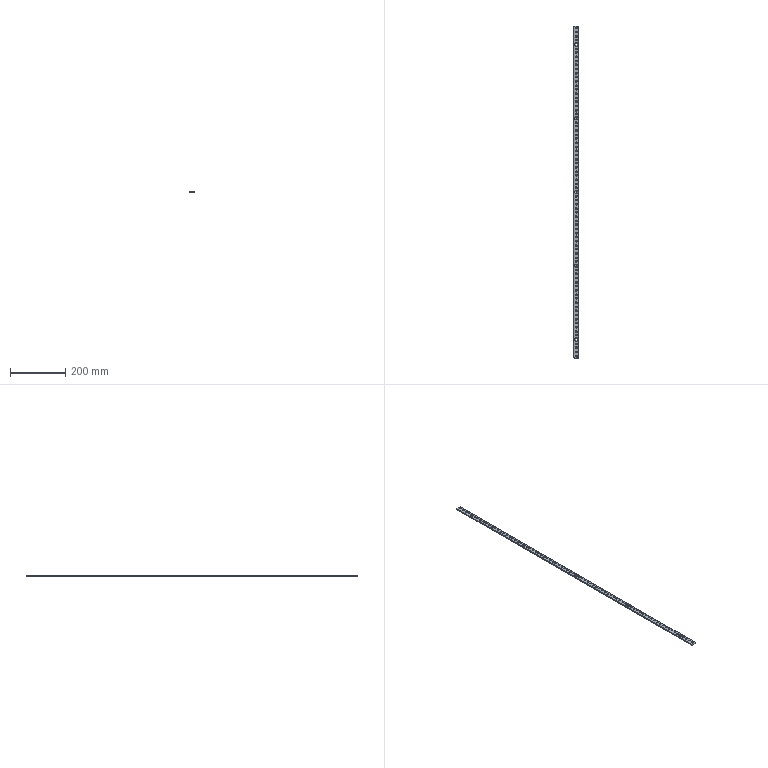CAM job | Mastercam | mm | 9 operations | part box 17.3 x 1200.15 x 6
1. Contour (Ramp) | 9 - 10 平铣刀
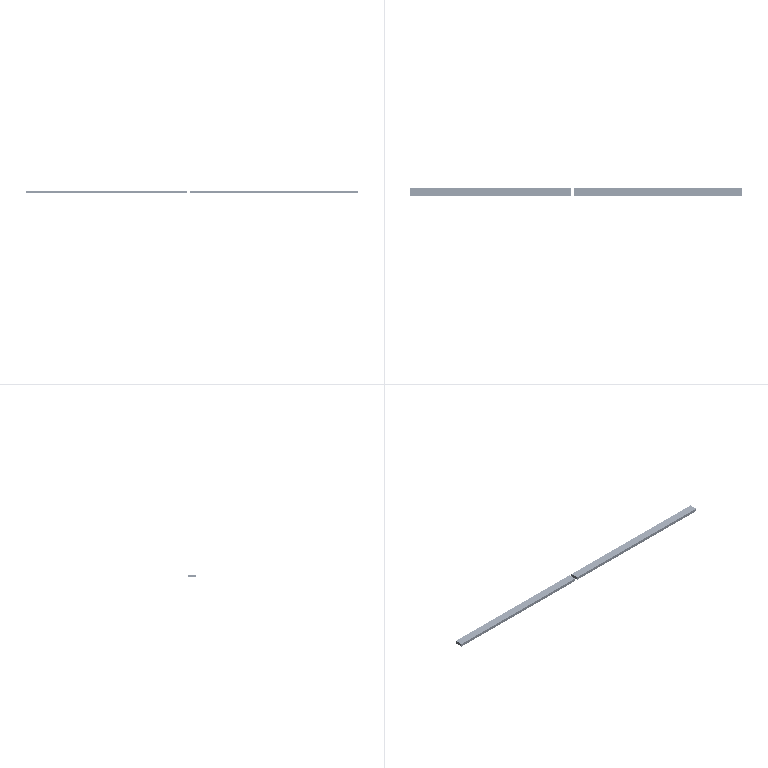2. Contour (2D) | 10 - 10 平铣刀
3. Drill/Counterbore | 7 - 6 倒角刀
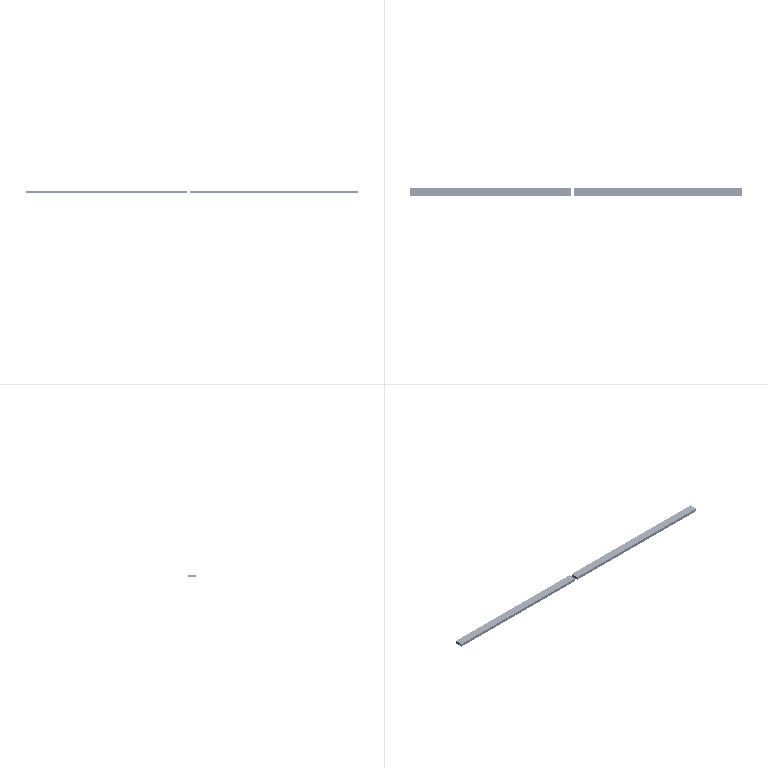4. Drill/Counterbore | 7 - 6 倒角刀
5. Contour (2D chamfer) | 7 - 6 倒角刀
6. Contour (2D chamfer) | 7 - 6 倒角刀
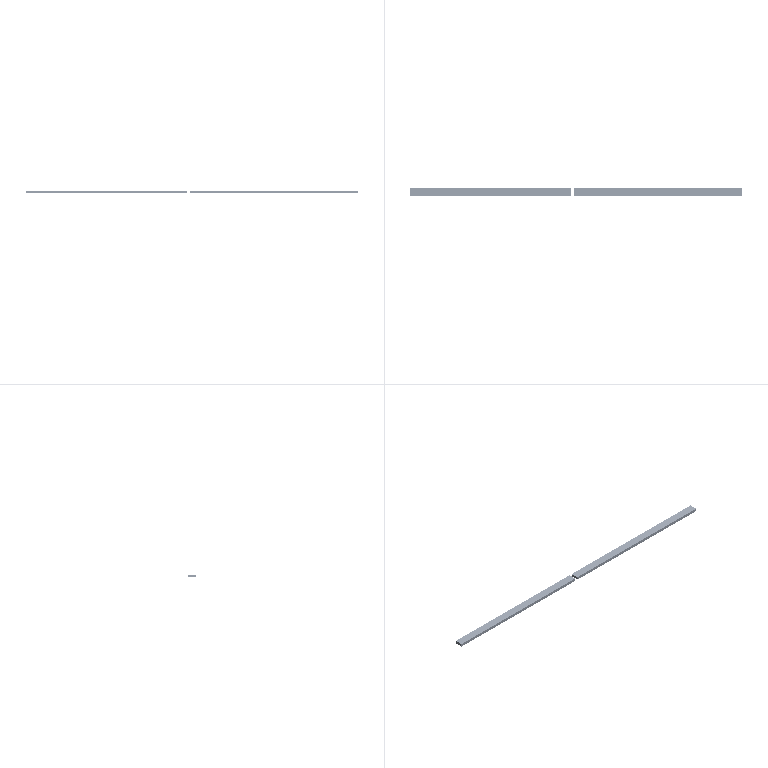7. Contour (Ramp) | 9 - 10 平铣刀
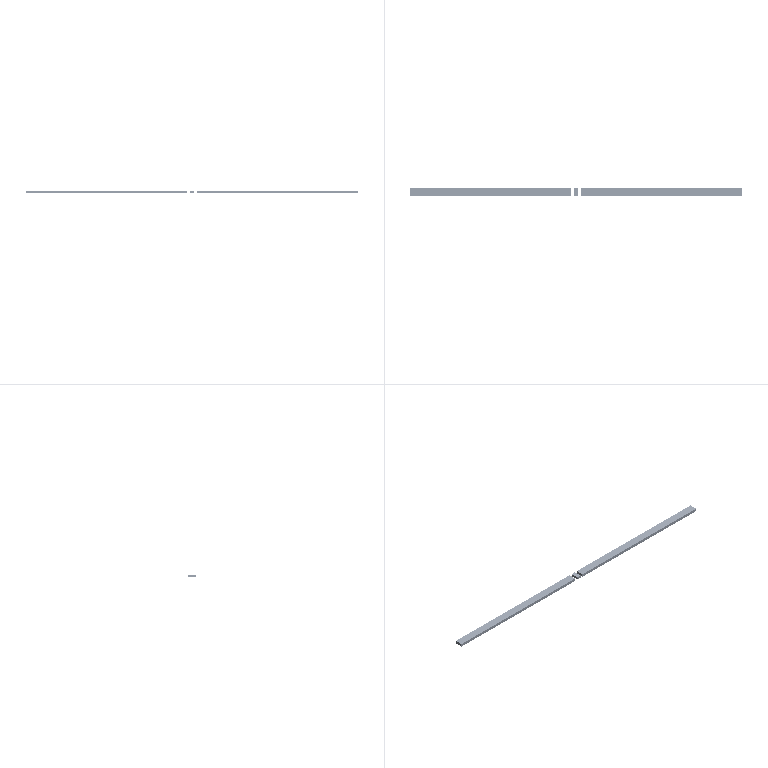8. Contour (2D) | 8 - 8 平铣刀
9. Contour (2D chamfer) | 7 - 6 倒角刀